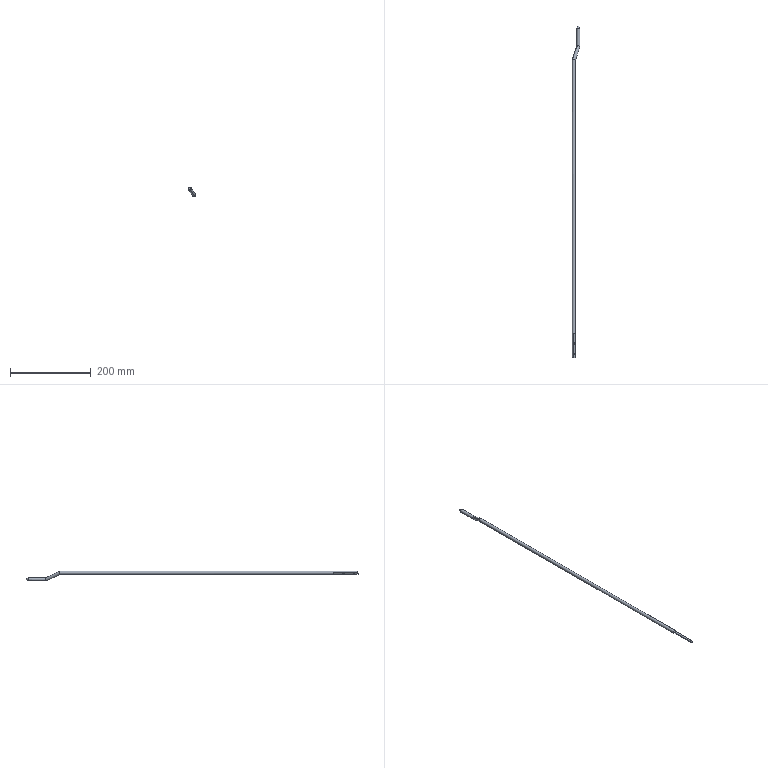Component | SolidWorks | UpperLockRod-1 | 1 solid | 18 faces | box 19.33 x 820.12 x 24.12 mm | volume 40012 mm3 | cylinder 10 | plane 6 | cone 2 | commonest cylinder face diameters 8 x6 4.2 x4
STEP:
#1=COLOUR_RGB('',0.7922,0.8196,0.9333);
#2=FILL_AREA_STYLE_COLOUR('',#1);
#3=FILL_AREA_STYLE('',(#2));
#4=SURFACE_STYLE_FILL_AREA(#3);
#5=SURFACE_SIDE_STYLE('',(#4));
#6=SURFACE_STYLE_USAGE(.BOTH.,#5);
#7=PRESENTATION_STYLE_ASSIGNMENT((#6));
#8=CARTESIAN_POINT('',(-12.605,2.873,84.686));
#9=VERTEX_POINT('',#8);
#10=CARTESIAN_POINT('',(-12.605,3.038,84.686));
#11=VERTEX_POINT('',#10);
#12=CARTESIAN_POINT('',(-12.605,2.956,84.686));
#13=DIRECTION('',(0.818,0.,0.5751));
#14=DIRECTION('',(0.,1.,0.));
#15=AXIS2_PLACEMENT_3D('',#12,#13,#14);
#16=CIRCLE('',#15,0.08268);
#17=EDGE_CURVE('',#9,#11,#16,.T.);
#18=ORIENTED_EDGE('',*,*,#17,.F.);
#19=CARTESIAN_POINT('',(-12.476,2.873,84.776));
#20=VERTEX_POINT('',#19);
#21=CARTESIAN_POINT('',(-14.408,2.873,83.418));
#22=DIRECTION('',(0.818,0.,0.5751));
#23=VECTOR('',#22,39.37);
#24=LINE('',#21,#23);
#25=EDGE_CURVE('',#9,#20,#24,.T.);
#26=ORIENTED_EDGE('',*,*,#25,.T.);
#27=CARTESIAN_POINT('',(-12.476,3.038,84.776));
#28=VERTEX_POINT('',#27);
#29=CARTESIAN_POINT('',(-12.476,2.956,84.776));
#30=DIRECTION('',(0.818,0.,0.5751));
#31=DIRECTION('',(0.,1.,0.));
#32=AXIS2_PLACEMENT_3D('',#29,#30,#31);
#33=CIRCLE('',#32,0.08268);
#34=EDGE_CURVE('',#20,#28,#33,.T.);
#35=ORIENTED_EDGE('',*,*,#34,.T.);
#36=CARTESIAN_POINT('',(-14.408,3.038,83.418));
#37=DIRECTION('',(0.818,0.,0.5751));
#38=VECTOR('',#37,39.37);
#39=LINE('',#36,#38);
#40=EDGE_CURVE('',#11,#28,#39,.T.);
#41=ORIENTED_EDGE('',*,*,#40,.F.);
#42=EDGE_LOOP('',(#18,#26,#35,#41));
#43=FACE_OUTER_BOUND('',#42,.T.);
#44=CARTESIAN_POINT('',(-14.408,2.956,83.418));
#45=DIRECTION('',(0.818,0.,0.5751));
#46=DIRECTION('',(0.,1.,0.));
#47=AXIS2_PLACEMENT_3D('',#44,#45,#46);
#48=CYLINDRICAL_SURFACE('',#47,0.08268);
#49=ADVANCED_FACE('',(#43),#48,.F.);
#50=CARTESIAN_POINT('',(-12.605,1.889,84.686));
#51=VERTEX_POINT('',#50);
#52=CARTESIAN_POINT('',(-12.605,2.054,84.686));
#53=VERTEX_POINT('',#52);
#54=CARTESIAN_POINT('',(-12.605,1.971,84.686));
#55=DIRECTION('',(0.818,0.,0.5751));
#56=DIRECTION('',(0.,1.,0.));
#57=AXIS2_PLACEMENT_3D('',#54,#55,#56);
#58=CIRCLE('',#57,0.08268);
#59=EDGE_CURVE('',#51,#53,#58,.T.);
#60=ORIENTED_EDGE('',*,*,#59,.F.);
#61=CARTESIAN_POINT('',(-12.476,1.889,84.776));
#62=VERTEX_POINT('',#61);
#63=CARTESIAN_POINT('',(-14.408,1.889,83.418));
#64=DIRECTION('',(0.818,0.,0.5751));
#65=VECTOR('',#64,39.37);
#66=LINE('',#63,#65);
#67=EDGE_CURVE('',#51,#62,#66,.T.);
#68=ORIENTED_EDGE('',*,*,#67,.T.);
#69=CARTESIAN_POINT('',(-12.476,2.054,84.776));
#70=VERTEX_POINT('',#69);
#71=CARTESIAN_POINT('',(-12.476,1.971,84.776));
#72=DIRECTION('',(0.818,0.,0.5751));
#73=DIRECTION('',(0.,1.,0.));
#74=AXIS2_PLACEMENT_3D('',#71,#72,#73);
#75=CIRCLE('',#74,0.08268);
#76=EDGE_CURVE('',#62,#70,#75,.T.);
#77=ORIENTED_EDGE('',*,*,#76,.T.);
#78=CARTESIAN_POINT('',(-14.408,2.054,83.418));
#79=DIRECTION('',(0.818,0.,0.5751));
#80=VECTOR('',#79,39.37);
#81=LINE('',#78,#80);
#82=EDGE_CURVE('',#53,#70,#81,.T.);
#83=ORIENTED_EDGE('',*,*,#82,.F.);
#84=EDGE_LOOP('',(#60,#68,#77,#83));
#85=FACE_OUTER_BOUND('',#84,.T.);
#86=CARTESIAN_POINT('',(-14.408,1.971,83.418));
#87=DIRECTION('',(0.818,0.,0.5751));
#88=DIRECTION('',(0.,1.,0.));
#89=AXIS2_PLACEMENT_3D('',#86,#87,#88);
#90=CYLINDRICAL_SURFACE('',#89,0.08268);
#91=ADVANCED_FACE('',(#85),#90,.F.);
#92=CARTESIAN_POINT('',(-12.11,33.866,84.085));
#93=VERTEX_POINT('',#92);
#94=CARTESIAN_POINT('',(-12.078,33.866,84.108));
#95=VERTEX_POINT('',#94);
#96=CARTESIAN_POINT('',(-12.094,33.866,84.097));
#97=DIRECTION('',(0.,1.,-0.));
#98=DIRECTION('',(-0.818,0.,-0.5751));
#99=AXIS2_PLACEMENT_3D('',#96,#97,#98);
#100=CIRCLE('',#99,0.01969);
#101=EDGE_CURVE('',#93,#95,#100,.T.);
#102=ORIENTED_EDGE('',*,*,#101,.F.);
#103=CARTESIAN_POINT('',(-12.223,33.63,84.006));
#104=VERTEX_POINT('',#103);
#105=CARTESIAN_POINT('',(-12.11,33.866,84.085));
#106=DIRECTION('',(-0.4122,-0.8638,-0.2898));
#107=VECTOR('',#106,39.37);
#108=LINE('',#105,#107);
#109=EDGE_CURVE('',#93,#104,#108,.T.);
#110=ORIENTED_EDGE('',*,*,#109,.T.);
#111=CARTESIAN_POINT('',(-11.966,33.63,84.187));
#112=VERTEX_POINT('',#111);
#113=CARTESIAN_POINT('',(-12.094,33.63,84.097));
#114=DIRECTION('',(-0.,-1.,0.));
#115=DIRECTION('',(-0.818,0.,-0.5751));
#116=AXIS2_PLACEMENT_3D('',#113,#114,#115);
#117=CIRCLE('',#116,0.1575);
#118=EDGE_CURVE('',#112,#104,#117,.T.);
#119=ORIENTED_EDGE('',*,*,#118,.F.);
#120=CARTESIAN_POINT('',(-12.078,33.866,84.108));
#121=DIRECTION('',(0.4122,-0.8638,0.2898));
#122=VECTOR('',#121,39.37);
#123=LINE('',#120,#122);
#124=EDGE_CURVE('',#95,#112,#123,.T.);
#125=ORIENTED_EDGE('',*,*,#124,.F.);
#126=EDGE_LOOP('',(#102,#110,#119,#125));
#127=FACE_OUTER_BOUND('',#126,.T.);
#128=CARTESIAN_POINT('',(-12.094,33.866,84.097));
#129=DIRECTION('',(-0.,-1.,0.));
#130=DIRECTION('',(0.818,0.,0.5751));
#131=AXIS2_PLACEMENT_3D('',#128,#129,#130);
#132=CONICAL_SURFACE('',#131,0.01969,0.5281);
#133=ADVANCED_FACE('',(#127),#132,.T.);
#134=CARTESIAN_POINT('',(-12.669,30.554,84.64));
#135=VERTEX_POINT('',#134);
#136=CARTESIAN_POINT('',(-12.631,30.596,84.86));
#137=VERTEX_POINT('',#136);
#138=CARTESIAN_POINT('',(-12.669,30.554,84.64));
#139=CARTESIAN_POINT('',(-12.722,30.579,84.716));
#140=CARTESIAN_POINT('',(-12.706,30.596,84.807));
#141=CARTESIAN_POINT('',(-12.631,30.596,84.86));
#142=(BOUNDED_CURVE()B_SPLINE_CURVE(3,(#138,#139,#140,#141),.UNSPECIFIED.,.F.,.F.)B_SPLINE_CURVE_WITH_KNOTS((4,4),(1.571,3.142),.UNSPECIFIED.)CURVE()GEOMETRIC_REPRESENTATION_ITEM()RATIONAL_B_SPLINE_CURVE((1.,0.8047,0.8047,1.))REPRESENTATION_ITEM(''));
#143=EDGE_CURVE('',#135,#137,#142,.T.);
#144=ORIENTED_EDGE('',*,*,#143,.F.);
#145=CARTESIAN_POINT('',(-12.669,3.94,84.64));
#146=VERTEX_POINT('',#145);
#147=CARTESIAN_POINT('',(-12.669,30.999,84.64));
#148=DIRECTION('',(-0.,-1.,0.));
#149=VECTOR('',#148,39.37);
#150=LINE('',#147,#149);
#151=EDGE_CURVE('',#135,#146,#150,.T.);
#152=ORIENTED_EDGE('',*,*,#151,.T.);
#153=CARTESIAN_POINT('',(-12.683,3.94,84.797));
#154=VERTEX_POINT('',#153);
#155=CARTESIAN_POINT('',(-12.54,3.94,84.731));
#156=DIRECTION('',(-0.,-1.,0.));
#157=DIRECTION('',(0.818,0.,0.5751));
#158=AXIS2_PLACEMENT_3D('',#155,#156,#157);
#159=CIRCLE('',#158,0.1575);
#160=EDGE_CURVE('',#154,#146,#159,.T.);
#161=ORIENTED_EDGE('',*,*,#160,.F.);
#162=CARTESIAN_POINT('',(-12.683,1.578,84.797));
#163=VERTEX_POINT('',#162);
#164=CARTESIAN_POINT('',(-12.683,3.94,84.797));
#165=DIRECTION('',(-0.,-1.,0.));
#166=VECTOR('',#165,39.37);
#167=LINE('',#164,#166);
#168=EDGE_CURVE('',#154,#163,#167,.T.);
#169=ORIENTED_EDGE('',*,*,#168,.T.);
#170=CARTESIAN_POINT('',(-12.554,1.578,84.888));
#171=VERTEX_POINT('',#170);
#172=CARTESIAN_POINT('',(-12.54,1.578,84.731));
#173=DIRECTION('',(0.,1.,-0.));
#174=DIRECTION('',(-0.818,-0.,-0.5751));
#175=AXIS2_PLACEMENT_3D('',#172,#173,#174);
#176=CIRCLE('',#175,0.1575);
#177=EDGE_CURVE('',#163,#171,#176,.T.);
#178=ORIENTED_EDGE('',*,*,#177,.T.);
#179=CARTESIAN_POINT('',(-12.554,3.94,84.888));
#180=VERTEX_POINT('',#179);
#181=CARTESIAN_POINT('',(-12.554,3.94,84.888));
#182=DIRECTION('',(-0.,-1.,0.));
#183=VECTOR('',#182,39.37);
#184=LINE('',#181,#183);
#185=EDGE_CURVE('',#180,#171,#184,.T.);
#186=ORIENTED_EDGE('',*,*,#185,.F.);
#187=CARTESIAN_POINT('',(-12.412,3.94,84.822));
#188=VERTEX_POINT('',#187);
#189=CARTESIAN_POINT('',(-12.54,3.94,84.731));
#190=DIRECTION('',(-0.,-1.,0.));
#191=DIRECTION('',(0.818,0.,0.5751));
#192=AXIS2_PLACEMENT_3D('',#189,#190,#191);
#193=CIRCLE('',#192,0.1575);
#194=EDGE_CURVE('',#188,#180,#193,.T.);
#195=ORIENTED_EDGE('',*,*,#194,.F.);
#196=CARTESIAN_POINT('',(-12.412,30.554,84.822));
#197=VERTEX_POINT('',#196);
#198=CARTESIAN_POINT('',(-12.412,30.999,84.822));
#199=DIRECTION('',(-0.,-1.,0.));
#200=VECTOR('',#199,39.37);
#201=LINE('',#198,#200);
#202=EDGE_CURVE('',#197,#188,#201,.T.);
#203=ORIENTED_EDGE('',*,*,#202,.F.);
#204=CARTESIAN_POINT('',(-12.631,30.596,84.86));
#205=CARTESIAN_POINT('',(-12.556,30.596,84.913));
#206=CARTESIAN_POINT('',(-12.465,30.579,84.897));
#207=CARTESIAN_POINT('',(-12.412,30.554,84.822));
#208=(BOUNDED_CURVE()B_SPLINE_CURVE(3,(#204,#205,#206,#207),.UNSPECIFIED.,.F.,.F.)B_SPLINE_CURVE_WITH_KNOTS((4,4),(3.142,4.712),.UNSPECIFIED.)CURVE()GEOMETRIC_REPRESENTATION_ITEM()RATIONAL_B_SPLINE_CURVE((1.,0.8047,0.8047,1.))REPRESENTATION_ITEM(''));
#209=EDGE_CURVE('',#137,#197,#208,.T.);
#210=ORIENTED_EDGE('',*,*,#209,.F.);
#211=EDGE_LOOP('',(#144,#152,#161,#169,#178,#186,#195,#203,#210));
#212=FACE_OUTER_BOUND('',#211,.T.);
#213=CARTESIAN_POINT('',(-12.54,30.999,84.731));
#214=DIRECTION('',(-0.,-1.,0.));
#215=DIRECTION('',(0.818,0.,0.5751));
#216=AXIS2_PLACEMENT_3D('',#213,#214,#215);
#217=CYLINDRICAL_SURFACE('',#216,0.1575);
#218=ADVANCED_FACE('',(#212),#217,.T.);
#219=ORIENTED_EDGE('',*,*,#209,.T.);
#220=CARTESIAN_POINT('',(-12.45,30.512,84.602));
#221=VERTEX_POINT('',#220);
#222=CARTESIAN_POINT('',(-12.412,30.554,84.822));
#223=CARTESIAN_POINT('',(-12.359,30.529,84.746));
#224=CARTESIAN_POINT('',(-12.374,30.512,84.655));
#225=CARTESIAN_POINT('',(-12.45,30.512,84.602));
#226=(BOUNDED_CURVE()B_SPLINE_CURVE(3,(#222,#223,#224,#225),.UNSPECIFIED.,.F.,.F.)B_SPLINE_CURVE_WITH_KNOTS((4,4),(4.712,6.283),.UNSPECIFIED.)CURVE()GEOMETRIC_REPRESENTATION_ITEM()RATIONAL_B_SPLINE_CURVE((1.,0.8047,0.8047,1.))REPRESENTATION_ITEM(''));
#227=EDGE_CURVE('',#197,#221,#226,.T.);
#228=ORIENTED_EDGE('',*,*,#227,.T.);
#229=CARTESIAN_POINT('',(-12.004,31.855,83.968));
#230=VERTEX_POINT('',#229);
#231=CARTESIAN_POINT('',(-12.462,30.475,84.619));
#232=DIRECTION('',(0.2876,0.866,-0.409));
#233=VECTOR('',#232,39.37);
#234=LINE('',#231,#233);
#235=EDGE_CURVE('',#221,#230,#234,.T.);
#236=ORIENTED_EDGE('',*,*,#235,.T.);
#237=CARTESIAN_POINT('',(-11.966,31.897,84.187));
#238=VERTEX_POINT('',#237);
#239=CARTESIAN_POINT('',(-12.004,31.855,83.968));
#240=CARTESIAN_POINT('',(-11.928,31.855,84.021));
#241=CARTESIAN_POINT('',(-11.912,31.873,84.112));
#242=CARTESIAN_POINT('',(-11.966,31.897,84.187));
#243=(BOUNDED_CURVE()B_SPLINE_CURVE(3,(#239,#240,#241,#242),.UNSPECIFIED.,.F.,.F.)B_SPLINE_CURVE_WITH_KNOTS((4,4),(-0.,1.571),.UNSPECIFIED.)CURVE()GEOMETRIC_REPRESENTATION_ITEM()RATIONAL_B_SPLINE_CURVE((1.,0.8047,0.8047,1.))REPRESENTATION_ITEM(''));
#244=EDGE_CURVE('',#230,#238,#243,.T.);
#245=ORIENTED_EDGE('',*,*,#244,.T.);
#246=CARTESIAN_POINT('',(-12.185,31.94,84.225));
#247=VERTEX_POINT('',#246);
#248=CARTESIAN_POINT('',(-11.966,31.897,84.187));
#249=CARTESIAN_POINT('',(-12.019,31.922,84.263));
#250=CARTESIAN_POINT('',(-12.109,31.94,84.278));
#251=CARTESIAN_POINT('',(-12.185,31.94,84.225));
#252=(BOUNDED_CURVE()B_SPLINE_CURVE(3,(#248,#249,#250,#251),.UNSPECIFIED.,.F.,.F.)B_SPLINE_CURVE_WITH_KNOTS((4,4),(1.571,3.142),.UNSPECIFIED.)CURVE()GEOMETRIC_REPRESENTATION_ITEM()RATIONAL_B_SPLINE_CURVE((1.,0.8047,0.8047,1.))REPRESENTATION_ITEM(''));
#253=EDGE_CURVE('',#238,#247,#252,.T.);
#254=ORIENTED_EDGE('',*,*,#253,.T.);
#255=CARTESIAN_POINT('',(-12.619,30.633,84.843));
#256=DIRECTION('',(0.2876,0.866,-0.409));
#257=VECTOR('',#256,39.37);
#258=LINE('',#255,#257);
#259=EDGE_CURVE('',#137,#247,#258,.T.);
#260=ORIENTED_EDGE('',*,*,#259,.F.);
#261=EDGE_LOOP('',(#219,#228,#236,#245,#254,#260));
#262=FACE_OUTER_BOUND('',#261,.T.);
#263=CARTESIAN_POINT('',(-12.54,30.554,84.731));
#264=DIRECTION('',(0.2876,0.866,-0.409));
#265=DIRECTION('',(-0.4981,0.5,0.7085));
#266=AXIS2_PLACEMENT_3D('',#263,#264,#265);
#267=CYLINDRICAL_SURFACE('',#266,0.1575);
#268=ADVANCED_FACE('',(#262),#267,.T.);
#269=ORIENTED_EDGE('',*,*,#253,.F.);
#270=CARTESIAN_POINT('',(-11.966,31.897,84.187));
#271=DIRECTION('',(0.,1.,-0.));
#272=VECTOR('',#271,39.37);
#273=LINE('',#270,#272);
#274=EDGE_CURVE('',#238,#112,#273,.T.);
#275=ORIENTED_EDGE('',*,*,#274,.T.);
#276=ORIENTED_EDGE('',*,*,#118,.T.);
#277=CARTESIAN_POINT('',(-12.223,31.897,84.006));
#278=VERTEX_POINT('',#277);
#279=CARTESIAN_POINT('',(-12.223,31.897,84.006));
#280=DIRECTION('',(0.,1.,-0.));
#281=VECTOR('',#280,39.37);
#282=LINE('',#279,#281);
#283=EDGE_CURVE('',#278,#104,#282,.T.);
#284=ORIENTED_EDGE('',*,*,#283,.F.);
#285=CARTESIAN_POINT('',(-12.185,31.94,84.225));
#286=CARTESIAN_POINT('',(-12.26,31.94,84.172));
#287=CARTESIAN_POINT('',(-12.276,31.922,84.081));
#288=CARTESIAN_POINT('',(-12.223,31.897,84.006));
#289=(BOUNDED_CURVE()B_SPLINE_CURVE(3,(#285,#286,#287,#288),.UNSPECIFIED.,.F.,.F.)B_SPLINE_CURVE_WITH_KNOTS((4,4),(3.142,4.712),.UNSPECIFIED.)CURVE()GEOMETRIC_REPRESENTATION_ITEM()RATIONAL_B_SPLINE_CURVE((1.,0.8047,0.8047,1.))REPRESENTATION_ITEM(''));
#290=EDGE_CURVE('',#247,#278,#289,.T.);
#291=ORIENTED_EDGE('',*,*,#290,.F.);
#292=EDGE_LOOP('',(#269,#275,#276,#284,#291));
#293=FACE_OUTER_BOUND('',#292,.T.);
#294=CARTESIAN_POINT('',(-12.094,31.897,84.097));
#295=DIRECTION('',(0.,1.,-0.));
#296=DIRECTION('',(-0.818,0.,-0.5751));
#297=AXIS2_PLACEMENT_3D('',#294,#295,#296);
#298=CYLINDRICAL_SURFACE('',#297,0.1575);
#299=ADVANCED_FACE('',(#293),#298,.T.);
#300=ORIENTED_EDGE('',*,*,#274,.F.);
#301=ORIENTED_EDGE('',*,*,#244,.F.);
#302=CARTESIAN_POINT('',(-12.223,31.897,84.006));
#303=CARTESIAN_POINT('',(-12.17,31.873,83.931));
#304=CARTESIAN_POINT('',(-12.079,31.855,83.915));
#305=CARTESIAN_POINT('',(-12.004,31.855,83.968));
#306=(BOUNDED_CURVE()B_SPLINE_CURVE(3,(#302,#303,#304,#305),.UNSPECIFIED.,.F.,.F.)B_SPLINE_CURVE_WITH_KNOTS((4,4),(4.712,6.283),.UNSPECIFIED.)CURVE()GEOMETRIC_REPRESENTATION_ITEM()RATIONAL_B_SPLINE_CURVE((1.,0.8047,0.8047,1.))REPRESENTATION_ITEM(''));
#307=EDGE_CURVE('',#278,#230,#306,.T.);
#308=ORIENTED_EDGE('',*,*,#307,.F.);
#309=ORIENTED_EDGE('',*,*,#283,.T.);
#310=CARTESIAN_POINT('',(-12.094,33.63,84.097));
#311=DIRECTION('',(-0.,-1.,0.));
#312=DIRECTION('',(-0.818,0.,-0.5751));
#313=AXIS2_PLACEMENT_3D('',#310,#311,#312);
#314=CIRCLE('',#313,0.1575);
#315=EDGE_CURVE('',#104,#112,#314,.T.);
#316=ORIENTED_EDGE('',*,*,#315,.T.);
#317=EDGE_LOOP('',(#300,#301,#308,#309,#316));
#318=FACE_OUTER_BOUND('',#317,.T.);
#319=CARTESIAN_POINT('',(-12.094,31.897,84.097));
#320=DIRECTION('',(0.,1.,-0.));
#321=DIRECTION('',(-0.818,0.,-0.5751));
#322=AXIS2_PLACEMENT_3D('',#319,#320,#321);
#323=CYLINDRICAL_SURFACE('',#322,0.1575);
#324=ADVANCED_FACE('',(#318),#323,.T.);
#325=ORIENTED_EDGE('',*,*,#235,.F.);
#326=CARTESIAN_POINT('',(-12.45,30.512,84.602));
#327=CARTESIAN_POINT('',(-12.525,30.512,84.549));
#328=CARTESIAN_POINT('',(-12.616,30.529,84.565));
#329=CARTESIAN_POINT('',(-12.669,30.554,84.64));
#330=(BOUNDED_CURVE()B_SPLINE_CURVE(3,(#326,#327,#328,#329),.UNSPECIFIED.,.F.,.F.)B_SPLINE_CURVE_WITH_KNOTS((4,4),(0.,1.571),.UNSPECIFIED.)CURVE()GEOMETRIC_REPRESENTATION_ITEM()RATIONAL_B_SPLINE_CURVE((1.,0.8047,0.8047,1.))REPRESENTATION_ITEM(''));
#331=EDGE_CURVE('',#221,#135,#330,.T.);
#332=ORIENTED_EDGE('',*,*,#331,.T.);
#333=ORIENTED_EDGE('',*,*,#143,.T.);
#334=ORIENTED_EDGE('',*,*,#259,.T.);
#335=ORIENTED_EDGE('',*,*,#290,.T.);
#336=ORIENTED_EDGE('',*,*,#307,.T.);
#337=EDGE_LOOP('',(#325,#332,#333,#334,#335,#336));
#338=FACE_OUTER_BOUND('',#337,.T.);
#339=CARTESIAN_POINT('',(-12.54,30.554,84.731));
#340=DIRECTION('',(0.2876,0.866,-0.409));
#341=DIRECTION('',(-0.4981,0.5,0.7085));
#342=AXIS2_PLACEMENT_3D('',#339,#340,#341);
#343=CYLINDRICAL_SURFACE('',#342,0.1575);
#344=ADVANCED_FACE('',(#338),#343,.T.);
#345=ORIENTED_EDGE('',*,*,#151,.F.);
#346=ORIENTED_EDGE('',*,*,#331,.F.);
#347=ORIENTED_EDGE('',*,*,#227,.F.);
#348=ORIENTED_EDGE('',*,*,#202,.T.);
#349=CARTESIAN_POINT('',(-12.398,3.94,84.665));
#350=VERTEX_POINT('',#349);
#351=CARTESIAN_POINT('',(-12.54,3.94,84.731));
#352=DIRECTION('',(-0.,-1.,0.));
#353=DIRECTION('',(0.818,0.,0.5751));
#354=AXIS2_PLACEMENT_3D('',#351,#352,#353);
#355=CIRCLE('',#354,0.1575);
#356=EDGE_CURVE('',#350,#188,#355,.T.);
#357=ORIENTED_EDGE('',*,*,#356,.F.);
#358=CARTESIAN_POINT('',(-12.398,1.578,84.665));
#359=VERTEX_POINT('',#358);
#360=CARTESIAN_POINT('',(-12.398,3.94,84.665));
#361=DIRECTION('',(-0.,-1.,0.));
#362=VECTOR('',#361,39.37);
#363=LINE('',#360,#362);
#364=EDGE_CURVE('',#350,#359,#363,.T.);
#365=ORIENTED_EDGE('',*,*,#364,.T.);
#366=CARTESIAN_POINT('',(-12.526,1.578,84.574));
#367=VERTEX_POINT('',#366);
#368=CARTESIAN_POINT('',(-12.54,1.578,84.731));
#369=DIRECTION('',(0.,1.,-0.));
#370=DIRECTION('',(-0.818,-0.,-0.5751));
#371=AXIS2_PLACEMENT_3D('',#368,#369,#370);
#372=CIRCLE('',#371,0.1575);
#373=EDGE_CURVE('',#359,#367,#372,.T.);
#374=ORIENTED_EDGE('',*,*,#373,.T.);
#375=CARTESIAN_POINT('',(-12.526,3.94,84.574));
#376=VERTEX_POINT('',#375);
#377=CARTESIAN_POINT('',(-12.526,3.94,84.574));
#378=DIRECTION('',(-0.,-1.,0.));
#379=VECTOR('',#378,39.37);
#380=LINE('',#377,#379);
#381=EDGE_CURVE('',#376,#367,#380,.T.);
#382=ORIENTED_EDGE('',*,*,#381,.F.);
#383=CARTESIAN_POINT('',(-12.54,3.94,84.731));
#384=DIRECTION('',(-0.,-1.,0.));
#385=DIRECTION('',(0.818,0.,0.5751));
#386=AXIS2_PLACEMENT_3D('',#383,#384,#385);
#387=CIRCLE('',#386,0.1575);
#388=EDGE_CURVE('',#146,#376,#387,.T.);
#389=ORIENTED_EDGE('',*,*,#388,.F.);
#390=EDGE_LOOP('',(#345,#346,#347,#348,#357,#365,#374,#382,#389));
#391=FACE_OUTER_BOUND('',#390,.T.);
#392=CARTESIAN_POINT('',(-12.54,30.999,84.731));
#393=DIRECTION('',(-0.,-1.,0.));
#394=DIRECTION('',(0.818,0.,0.5751));
#395=AXIS2_PLACEMENT_3D('',#392,#393,#394);
#396=CYLINDRICAL_SURFACE('',#395,0.1575);
#397=ADVANCED_FACE('',(#391),#396,.T.);
#398=ORIENTED_EDGE('',*,*,#177,.F.);
#399=CARTESIAN_POINT('',(-12.683,1.578,84.797));
#400=DIRECTION('',(-0.5751,0.,0.818));
#401=VECTOR('',#400,39.37);
#402=LINE('',#399,#401);
#403=EDGE_CURVE('',#367,#163,#402,.T.);
#404=ORIENTED_EDGE('',*,*,#403,.F.);
#405=ORIENTED_EDGE('',*,*,#373,.F.);
#406=CARTESIAN_POINT('',(-12.554,1.578,84.888));
#407=DIRECTION('',(0.5751,-0.,-0.818));
#408=VECTOR('',#407,39.37);
#409=LINE('',#406,#408);
#410=EDGE_CURVE('',#171,#359,#409,.T.);
#411=ORIENTED_EDGE('',*,*,#410,.F.);
#412=EDGE_LOOP('',(#398,#404,#405,#411));
#413=FACE_OUTER_BOUND('',#412,.T.);
#414=CARTESIAN_POINT('',(-12.54,1.578,84.731));
#415=DIRECTION('',(0.,1.,-0.));
#416=DIRECTION('',(-0.818,-0.,-0.5751));
#417=AXIS2_PLACEMENT_3D('',#414,#415,#416);
#418=PLANE('',#417);
#419=ADVANCED_FACE('',(#413),#418,.F.);
#420=CARTESIAN_POINT('',(-12.094,33.866,84.097));
#421=DIRECTION('',(0.,1.,-0.));
#422=DIRECTION('',(-0.818,0.,-0.5751));
#423=AXIS2_PLACEMENT_3D('',#420,#421,#422);
#424=CIRCLE('',#423,0.01969);
#425=EDGE_CURVE('',#95,#93,#424,.T.);
#426=ORIENTED_EDGE('',*,*,#425,.T.);
#427=ORIENTED_EDGE('',*,*,#101,.T.);
#428=EDGE_LOOP('',(#426,#427));
#429=FACE_OUTER_BOUND('',#428,.T.);
#430=CARTESIAN_POINT('',(-12.094,33.866,84.097));
#431=DIRECTION('',(0.,1.,-0.));
#432=DIRECTION('',(-0.818,-0.,-0.5751));
#433=AXIS2_PLACEMENT_3D('',#430,#431,#432);
#434=PLANE('',#433);
#435=ADVANCED_FACE('',(#429),#434,.T.);
#436=ORIENTED_EDGE('',*,*,#109,.F.);
#437=ORIENTED_EDGE('',*,*,#425,.F.);
#438=ORIENTED_EDGE('',*,*,#124,.T.);
#439=ORIENTED_EDGE('',*,*,#315,.F.);
#440=EDGE_LOOP('',(#436,#437,#438,#439));
#441=FACE_OUTER_BOUND('',#440,.T.);
#442=CARTESIAN_POINT('',(-12.094,33.866,84.097));
#443=DIRECTION('',(-0.,-1.,0.));
#444=DIRECTION('',(0.818,0.,0.5751));
#445=AXIS2_PLACEMENT_3D('',#442,#443,#444);
#446=CONICAL_SURFACE('',#445,0.01969,0.5281);
#447=ADVANCED_FACE('',(#441),#446,.T.);
#448=CARTESIAN_POINT('',(-12.476,2.956,84.776));
#449=DIRECTION('',(0.818,0.,0.5751));
#450=DIRECTION('',(0.,1.,0.));
#451=AXIS2_PLACEMENT_3D('',#448,#449,#450);
#452=CIRCLE('',#451,0.08268);
#453=EDGE_CURVE('',#28,#20,#452,.T.);
#454=ORIENTED_EDGE('',*,*,#453,.F.);
#455=ORIENTED_EDGE('',*,*,#34,.F.);
#456=EDGE_LOOP('',(#454,#455));
#457=FACE_BOUND('',#456,.T.);
#458=CARTESIAN_POINT('',(-12.476,1.971,84.776));
#459=DIRECTION('',(0.818,0.,0.5751));
#460=DIRECTION('',(0.,1.,0.));
#461=AXIS2_PLACEMENT_3D('',#458,#459,#460);
#462=CIRCLE('',#461,0.08268);
#463=EDGE_CURVE('',#70,#62,#462,.T.);
#464=ORIENTED_EDGE('',*,*,#463,.F.);
#465=ORIENTED_EDGE('',*,*,#76,.F.);
#466=EDGE_LOOP('',(#464,#465));
#467=FACE_BOUND('',#466,.T.);
#468=ORIENTED_EDGE('',*,*,#410,.T.);
#469=ORIENTED_EDGE('',*,*,#364,.F.);
#470=CARTESIAN_POINT('',(-12.554,3.94,84.888));
#471=DIRECTION('',(0.5751,-0.,-0.818));
#472=VECTOR('',#471,39.37);
#473=LINE('',#470,#472);
#474=EDGE_CURVE('',#180,#350,#473,.T.);
#475=ORIENTED_EDGE('',*,*,#474,.F.);
#476=ORIENTED_EDGE('',*,*,#185,.T.);
#477=EDGE_LOOP('',(#468,#469,#475,#476));
#478=FACE_OUTER_BOUND('',#477,.T.);
#479=CARTESIAN_POINT('',(-12.554,3.94,84.888));
#480=DIRECTION('',(-0.818,-0.,-0.5751));
#481=DIRECTION('',(-0.,-1.,0.));
#482=AXIS2_PLACEMENT_3D('',#479,#480,#481);
#483=PLANE('',#482);
#484=ADVANCED_FACE('',(#457,#467,#478),#483,.F.);
#485=ORIENTED_EDGE('',*,*,#356,.T.);
#486=ORIENTED_EDGE('',*,*,#194,.T.);
#487=ORIENTED_EDGE('',*,*,#474,.T.);
#488=EDGE_LOOP('',(#485,#486,#487));
#489=FACE_OUTER_BOUND('',#488,.T.);
#490=CARTESIAN_POINT('',(-12.54,3.94,84.731));
#491=DIRECTION('',(-0.,-1.,0.));
#492=DIRECTION('',(0.818,0.,0.5751));
#493=AXIS2_PLACEMENT_3D('',#490,#491,#492);
#494=PLANE('',#493);
#495=ADVANCED_FACE('',(#489),#494,.T.);
#496=CARTESIAN_POINT('',(-12.605,2.956,84.686));
#497=DIRECTION('',(0.818,0.,0.5751));
#498=DIRECTION('',(0.,1.,0.));
#499=AXIS2_PLACEMENT_3D('',#496,#497,#498);
#500=CIRCLE('',#499,0.08268);
#501=EDGE_CURVE('',#11,#9,#500,.T.);
#502=ORIENTED_EDGE('',*,*,#501,.T.);
#503=ORIENTED_EDGE('',*,*,#17,.T.);
#504=EDGE_LOOP('',(#502,#503));
#505=FACE_BOUND('',#504,.T.);
#506=CARTESIAN_POINT('',(-12.605,1.971,84.686));
#507=DIRECTION('',(0.818,0.,0.5751));
#508=DIRECTION('',(0.,1.,0.));
#509=AXIS2_PLACEMENT_3D('',#506,#507,#508);
#510=CIRCLE('',#509,0.08268);
#511=EDGE_CURVE('',#53,#51,#510,.T.);
#512=ORIENTED_EDGE('',*,*,#511,.T.);
#513=ORIENTED_EDGE('',*,*,#59,.T.);
#514=EDGE_LOOP('',(#512,#513));
#515=FACE_BOUND('',#514,.T.);
#516=ORIENTED_EDGE('',*,*,#403,.T.);
#517=ORIENTED_EDGE('',*,*,#168,.F.);
#518=CARTESIAN_POINT('',(-12.683,3.94,84.797));
#519=DIRECTION('',(-0.5751,0.,0.818));
#520=VECTOR('',#519,39.37);
#521=LINE('',#518,#520);
#522=EDGE_CURVE('',#376,#154,#521,.T.);
#523=ORIENTED_EDGE('',*,*,#522,.F.);
#524=ORIENTED_EDGE('',*,*,#381,.T.);
#525=EDGE_LOOP('',(#516,#517,#523,#524));
#526=FACE_OUTER_BOUND('',#525,.T.);
#527=CARTESIAN_POINT('',(-12.683,3.94,84.797));
#528=DIRECTION('',(0.818,0.,0.5751));
#529=DIRECTION('',(0.,1.,-0.));
#530=AXIS2_PLACEMENT_3D('',#527,#528,#529);
#531=PLANE('',#530);
#532=ADVANCED_FACE('',(#505,#515,#526),#531,.F.);
#533=ORIENTED_EDGE('',*,*,#160,.T.);
#534=ORIENTED_EDGE('',*,*,#388,.T.);
#535=ORIENTED_EDGE('',*,*,#522,.T.);
#536=EDGE_LOOP('',(#533,#534,#535));
#537=FACE_OUTER_BOUND('',#536,.T.);
#538=CARTESIAN_POINT('',(-12.54,3.94,84.731));
#539=DIRECTION('',(-0.,-1.,0.));
#540=DIRECTION('',(0.818,0.,0.5751));
#541=AXIS2_PLACEMENT_3D('',#538,#539,#540);
#542=PLANE('',#541);
#543=ADVANCED_FACE('',(#537),#542,.T.);
#544=ORIENTED_EDGE('',*,*,#67,.F.);
#545=ORIENTED_EDGE('',*,*,#511,.F.);
#546=ORIENTED_EDGE('',*,*,#82,.T.);
#547=ORIENTED_EDGE('',*,*,#463,.T.);
#548=EDGE_LOOP('',(#544,#545,#546,#547));
#549=FACE_OUTER_BOUND('',#548,.T.);
#550=CARTESIAN_POINT('',(-14.408,1.971,83.418));
#551=DIRECTION('',(0.818,0.,0.5751));
#552=DIRECTION('',(0.,1.,0.));
#553=AXIS2_PLACEMENT_3D('',#550,#551,#552);
#554=CYLINDRICAL_SURFACE('',#553,0.08268);
#555=ADVANCED_FACE('',(#549),#554,.F.);
#556=ORIENTED_EDGE('',*,*,#25,.F.);
#557=ORIENTED_EDGE('',*,*,#501,.F.);
#558=ORIENTED_EDGE('',*,*,#40,.T.);
#559=ORIENTED_EDGE('',*,*,#453,.T.);
#560=EDGE_LOOP('',(#556,#557,#558,#559));
#561=FACE_OUTER_BOUND('',#560,.T.);
#562=CARTESIAN_POINT('',(-14.408,2.956,83.418));
#563=DIRECTION('',(0.818,0.,0.5751));
#564=DIRECTION('',(0.,1.,0.));
#565=AXIS2_PLACEMENT_3D('',#562,#563,#564);
#566=CYLINDRICAL_SURFACE('',#565,0.08268);
#567=ADVANCED_FACE('',(#561),#566,.F.);
#568=CLOSED_SHELL('',(#49,#91,#133,#218,#268,#299,#324,#344,#397,#419,#435,#447,#484,#495,#532,#543,#555,#567));
#569=MANIFOLD_SOLID_BREP('',#568);
#570=STYLED_ITEM('',(#7),#569);
#571=(LENGTH_UNIT()NAMED_UNIT(*)SI_UNIT($,.METRE.));
#572=LENGTH_MEASURE_WITH_UNIT(LENGTH_MEASURE(0.0254),#571);
#573=DIMENSIONAL_EXPONENTS(1.,0.,0.,0.,0.,0.,0.);
#574=(CONVERSION_BASED_UNIT('',#572)LENGTH_UNIT()NAMED_UNIT(#573));
#575=UNCERTAINTY_MEASURE_WITH_UNIT(LENGTH_MEASURE(0.00001),#574,'','');
#576=(NAMED_UNIT(*)PLANE_ANGLE_UNIT()SI_UNIT($,.RADIAN.));
#577=(NAMED_UNIT(*)SI_UNIT($,.STERADIAN.)SOLID_ANGLE_UNIT());
#578=(GEOMETRIC_REPRESENTATION_CONTEXT(3)GLOBAL_UNCERTAINTY_ASSIGNED_CONTEXT((#575))GLOBAL_UNIT_ASSIGNED_CONTEXT((#574,#576,#577))REPRESENTATION_CONTEXT('',''));
#579=MECHANICAL_DESIGN_GEOMETRIC_PRESENTATION_REPRESENTATION('',(#570),#578);
#580=CARTESIAN_POINT('',(0.,0.,0.));
#581=DIRECTION('',(0.,0.,1.));
#582=DIRECTION('',(1.,0.,0.));
#583=AXIS2_PLACEMENT_3D('',#580,#581,#582);
#584=(LENGTH_UNIT()NAMED_UNIT(*)SI_UNIT($,.METRE.));
#585=LENGTH_MEASURE_WITH_UNIT(LENGTH_MEASURE(0.0254),#584);
#586=DIMENSIONAL_EXPONENTS(1.,0.,0.,0.,0.,0.,0.);
#587=(CONVERSION_BASED_UNIT('',#585)LENGTH_UNIT()NAMED_UNIT(#586));
#588=UNCERTAINTY_MEASURE_WITH_UNIT(LENGTH_MEASURE(0.00001),#587,'','');
#589=(NAMED_UNIT(*)PLANE_ANGLE_UNIT()SI_UNIT($,.RADIAN.));
#590=(NAMED_UNIT(*)SI_UNIT($,.STERADIAN.)SOLID_ANGLE_UNIT());
#591=(GEOMETRIC_REPRESENTATION_CONTEXT(3)GLOBAL_UNCERTAINTY_ASSIGNED_CONTEXT((#588))GLOBAL_UNIT_ASSIGNED_CONTEXT((#587,#589,#590))REPRESENTATION_CONTEXT('',''));
#592=ADVANCED_BREP_SHAPE_REPRESENTATION('',(#569,#583),#591);
#593=PRESENTATION_LAYER_ASSIGNMENT('','',(#570));